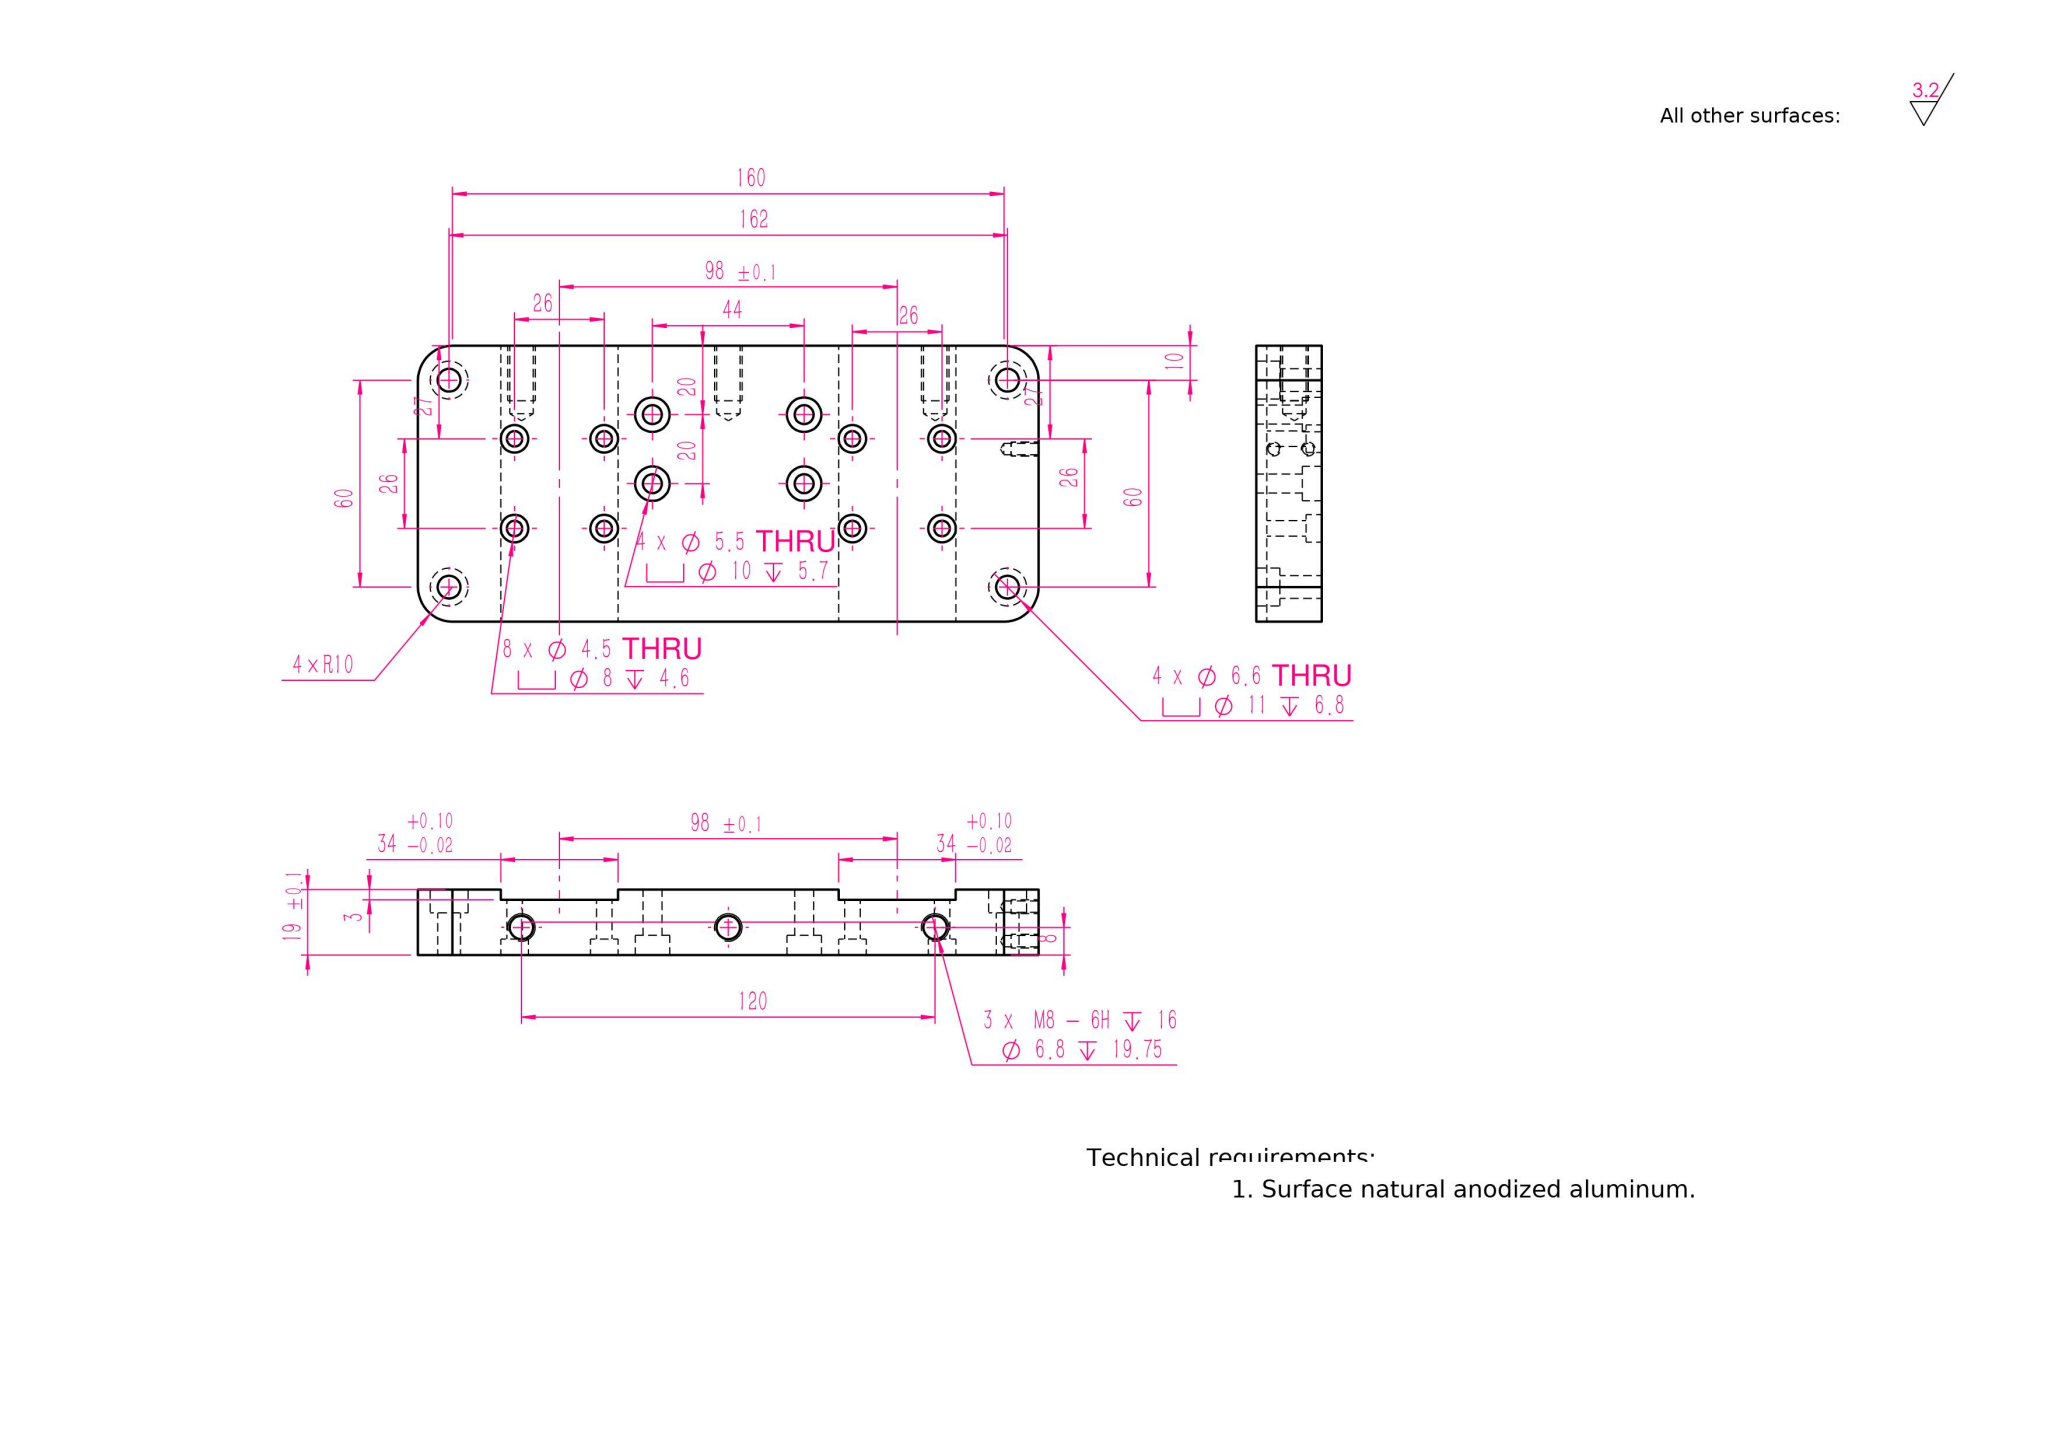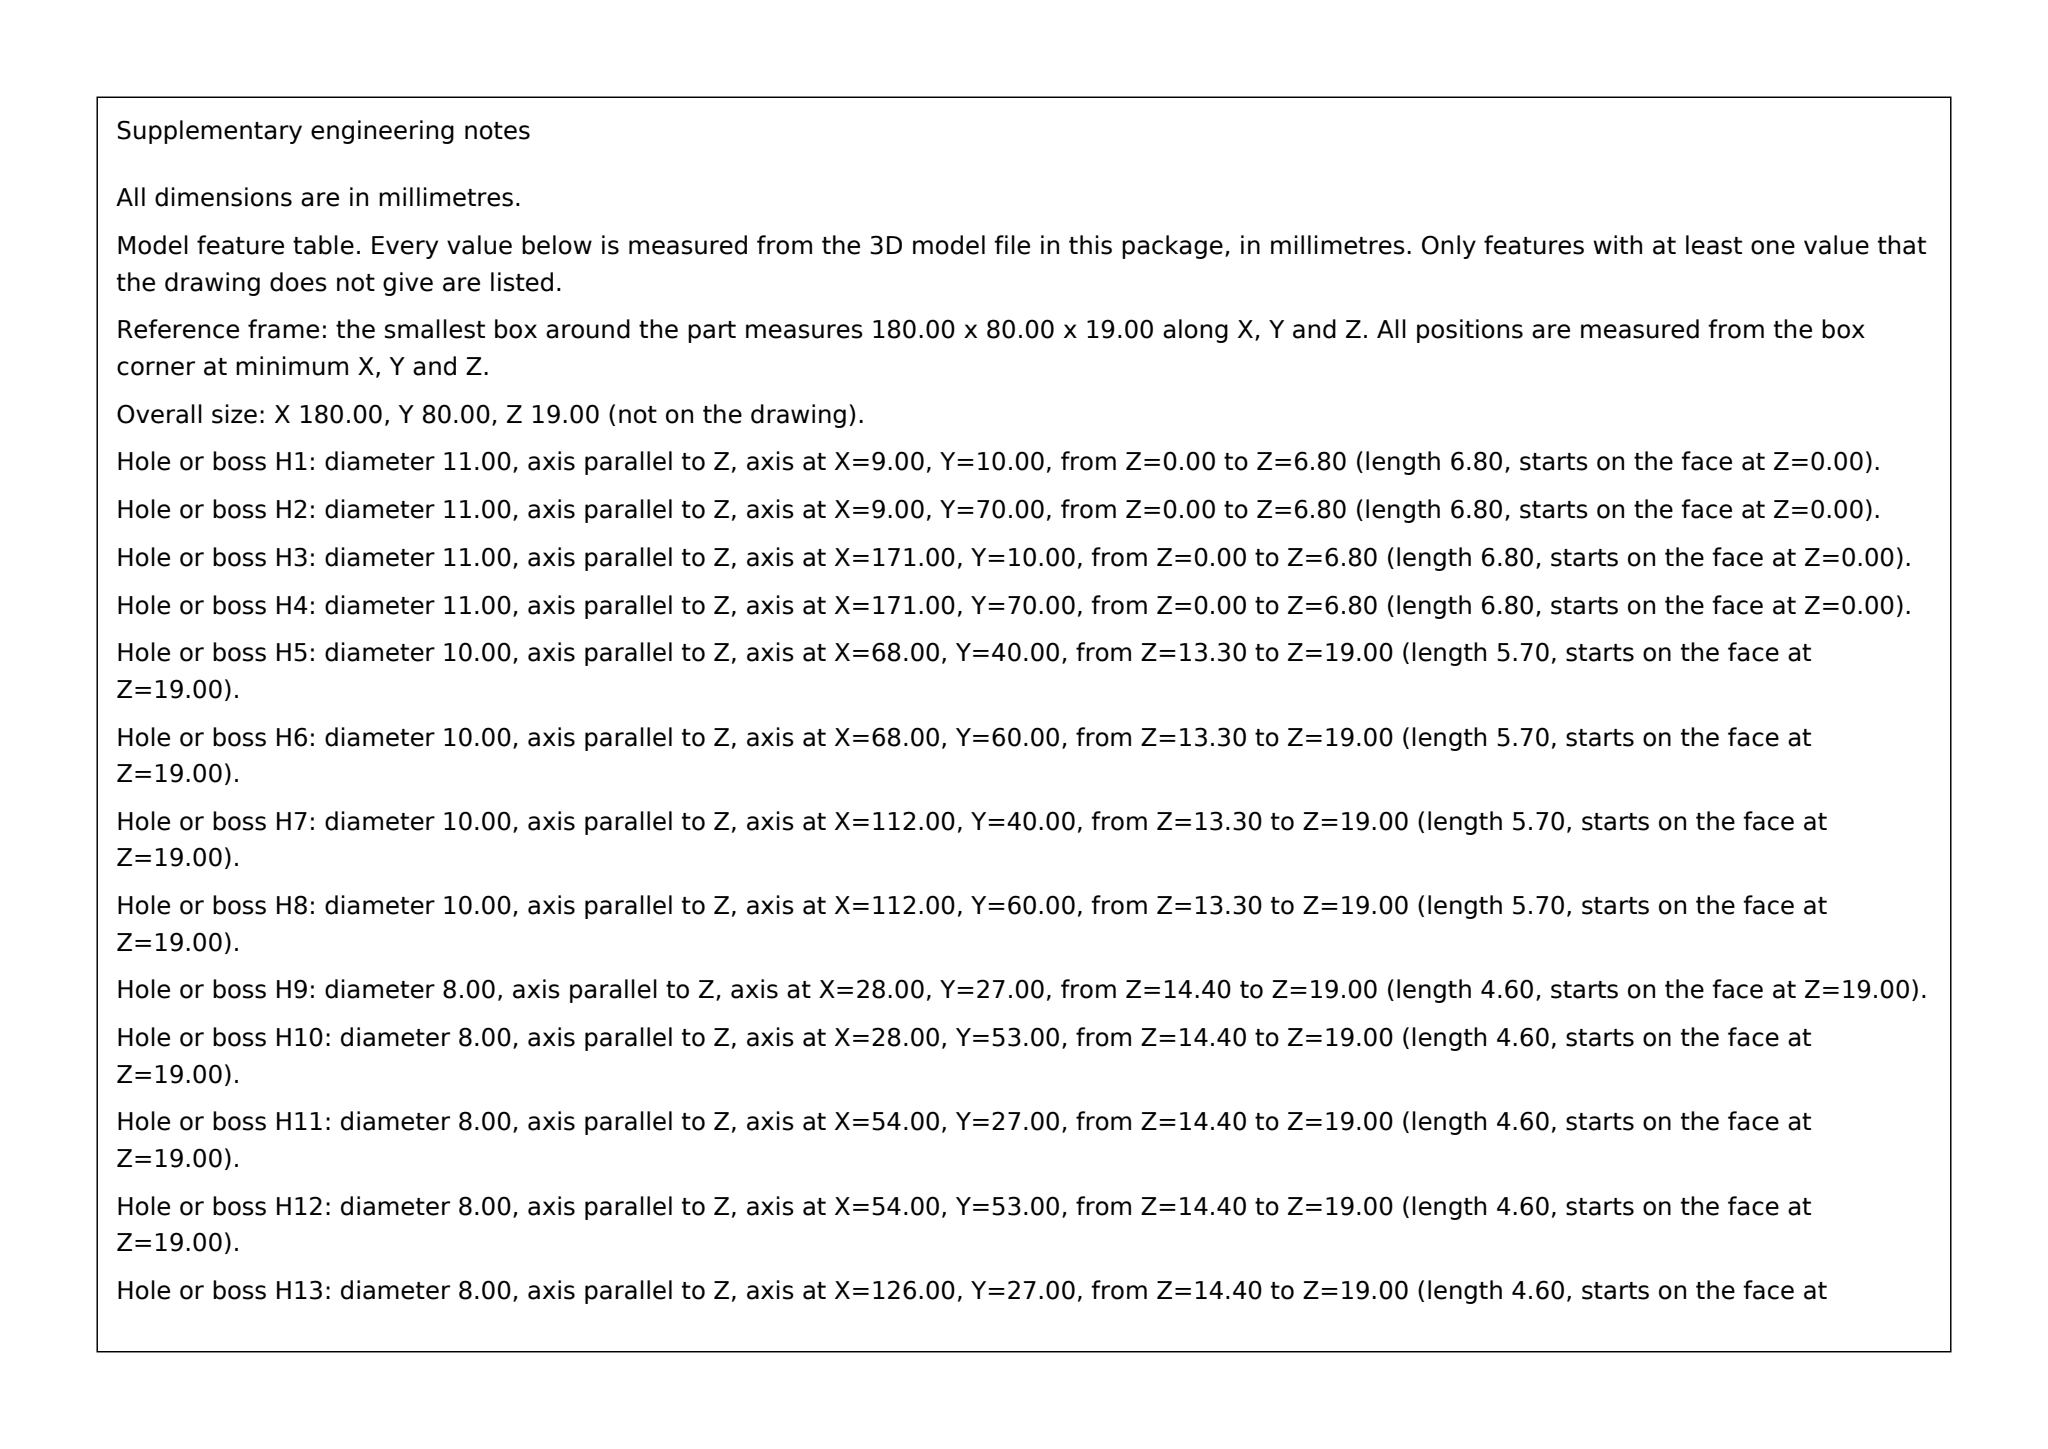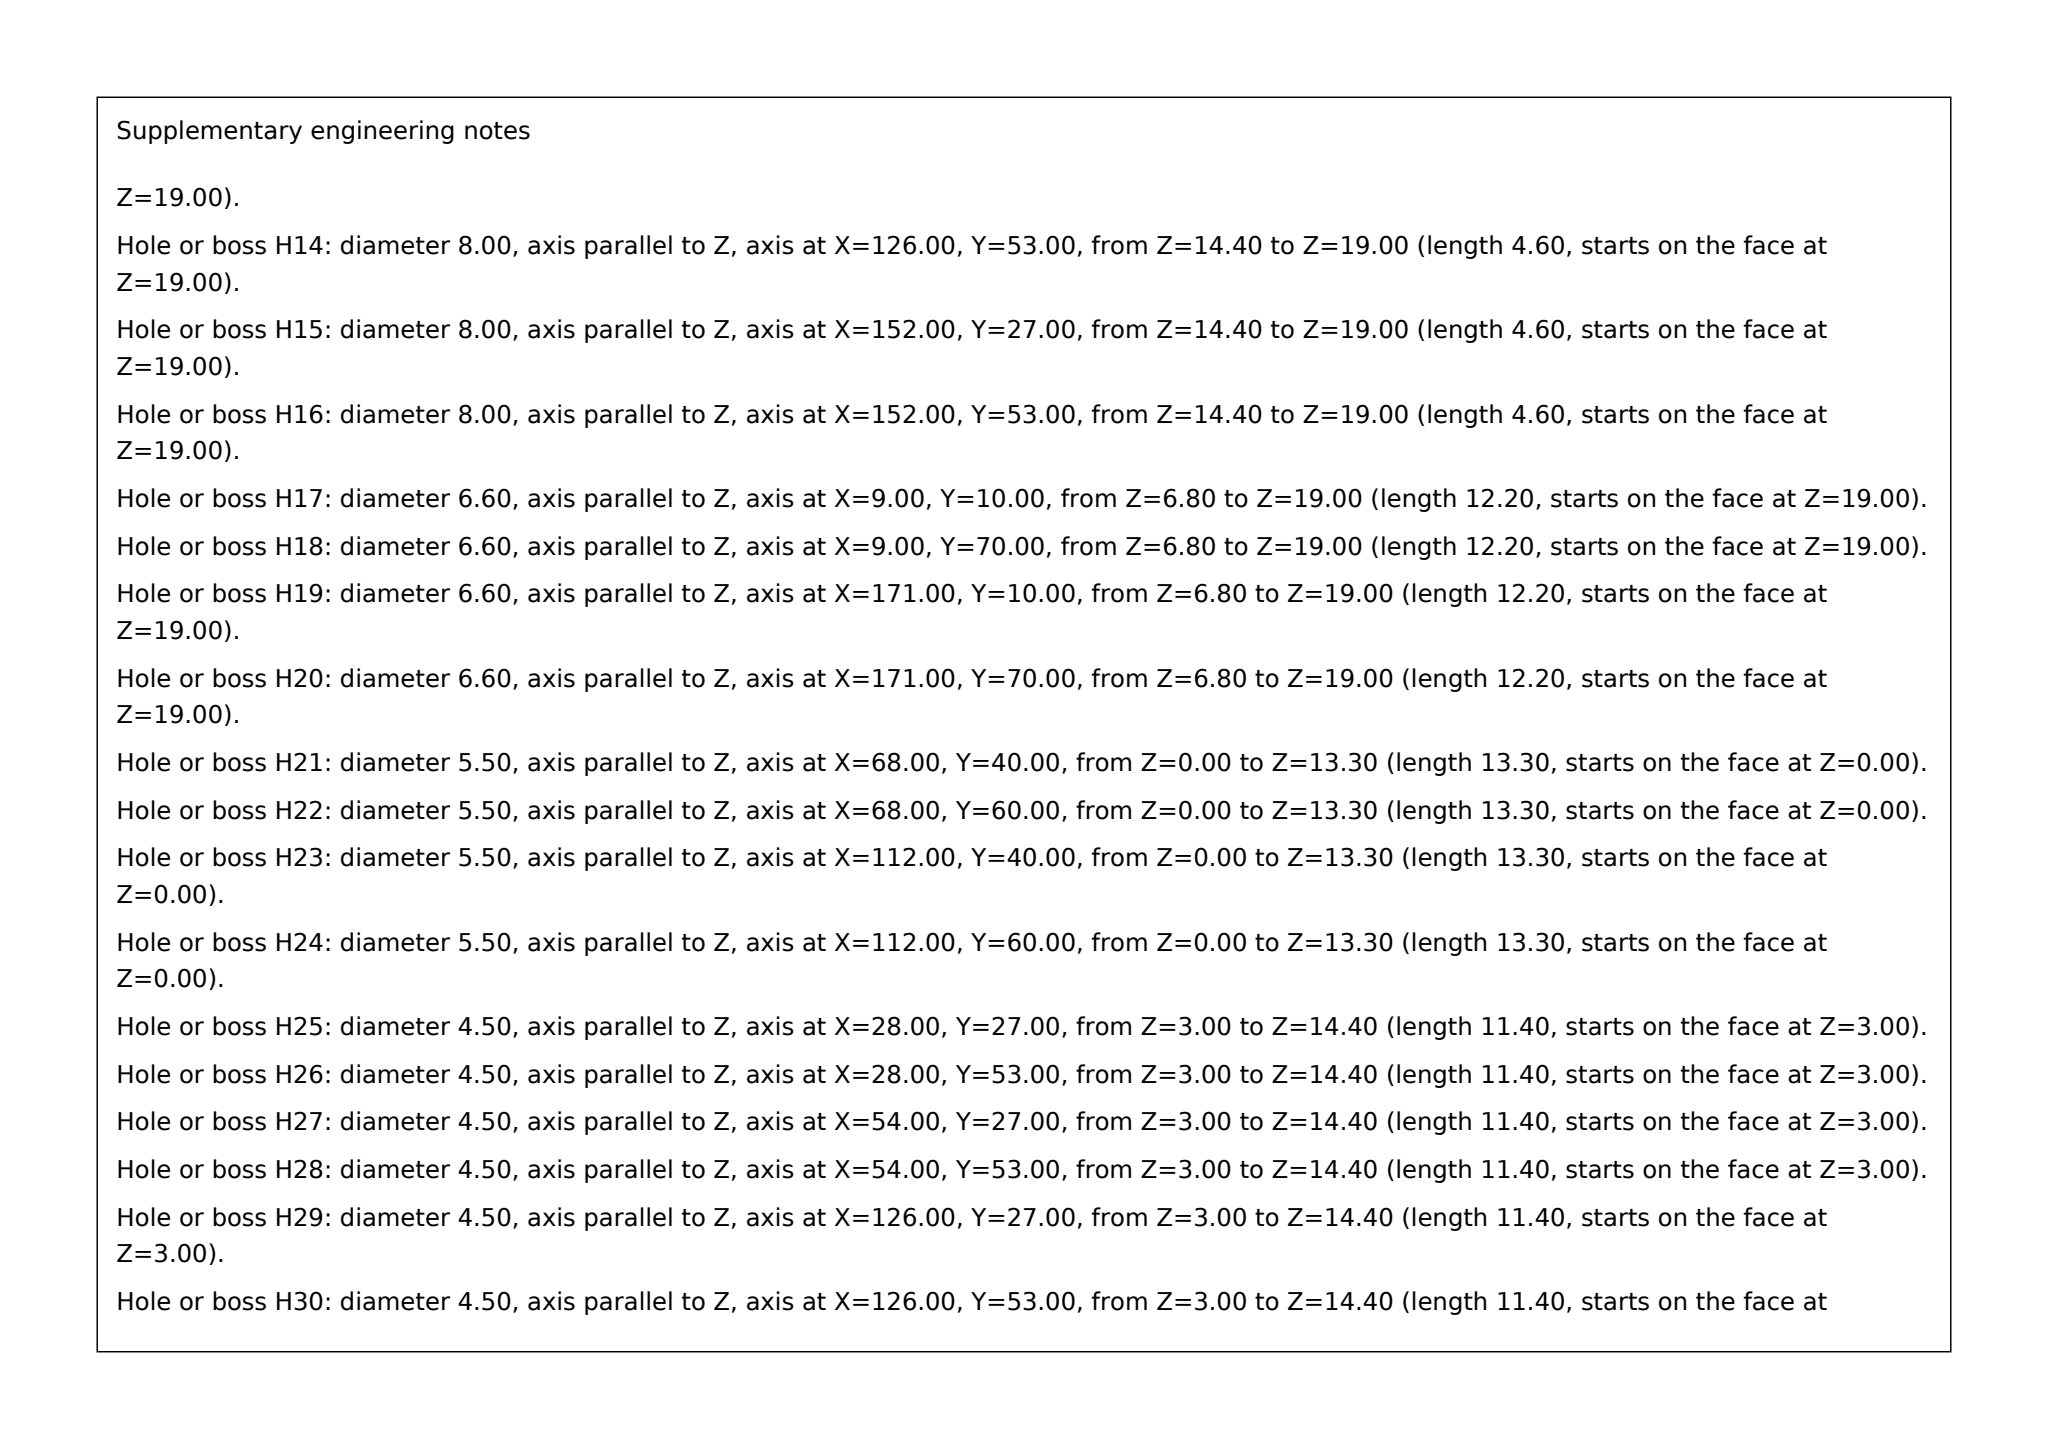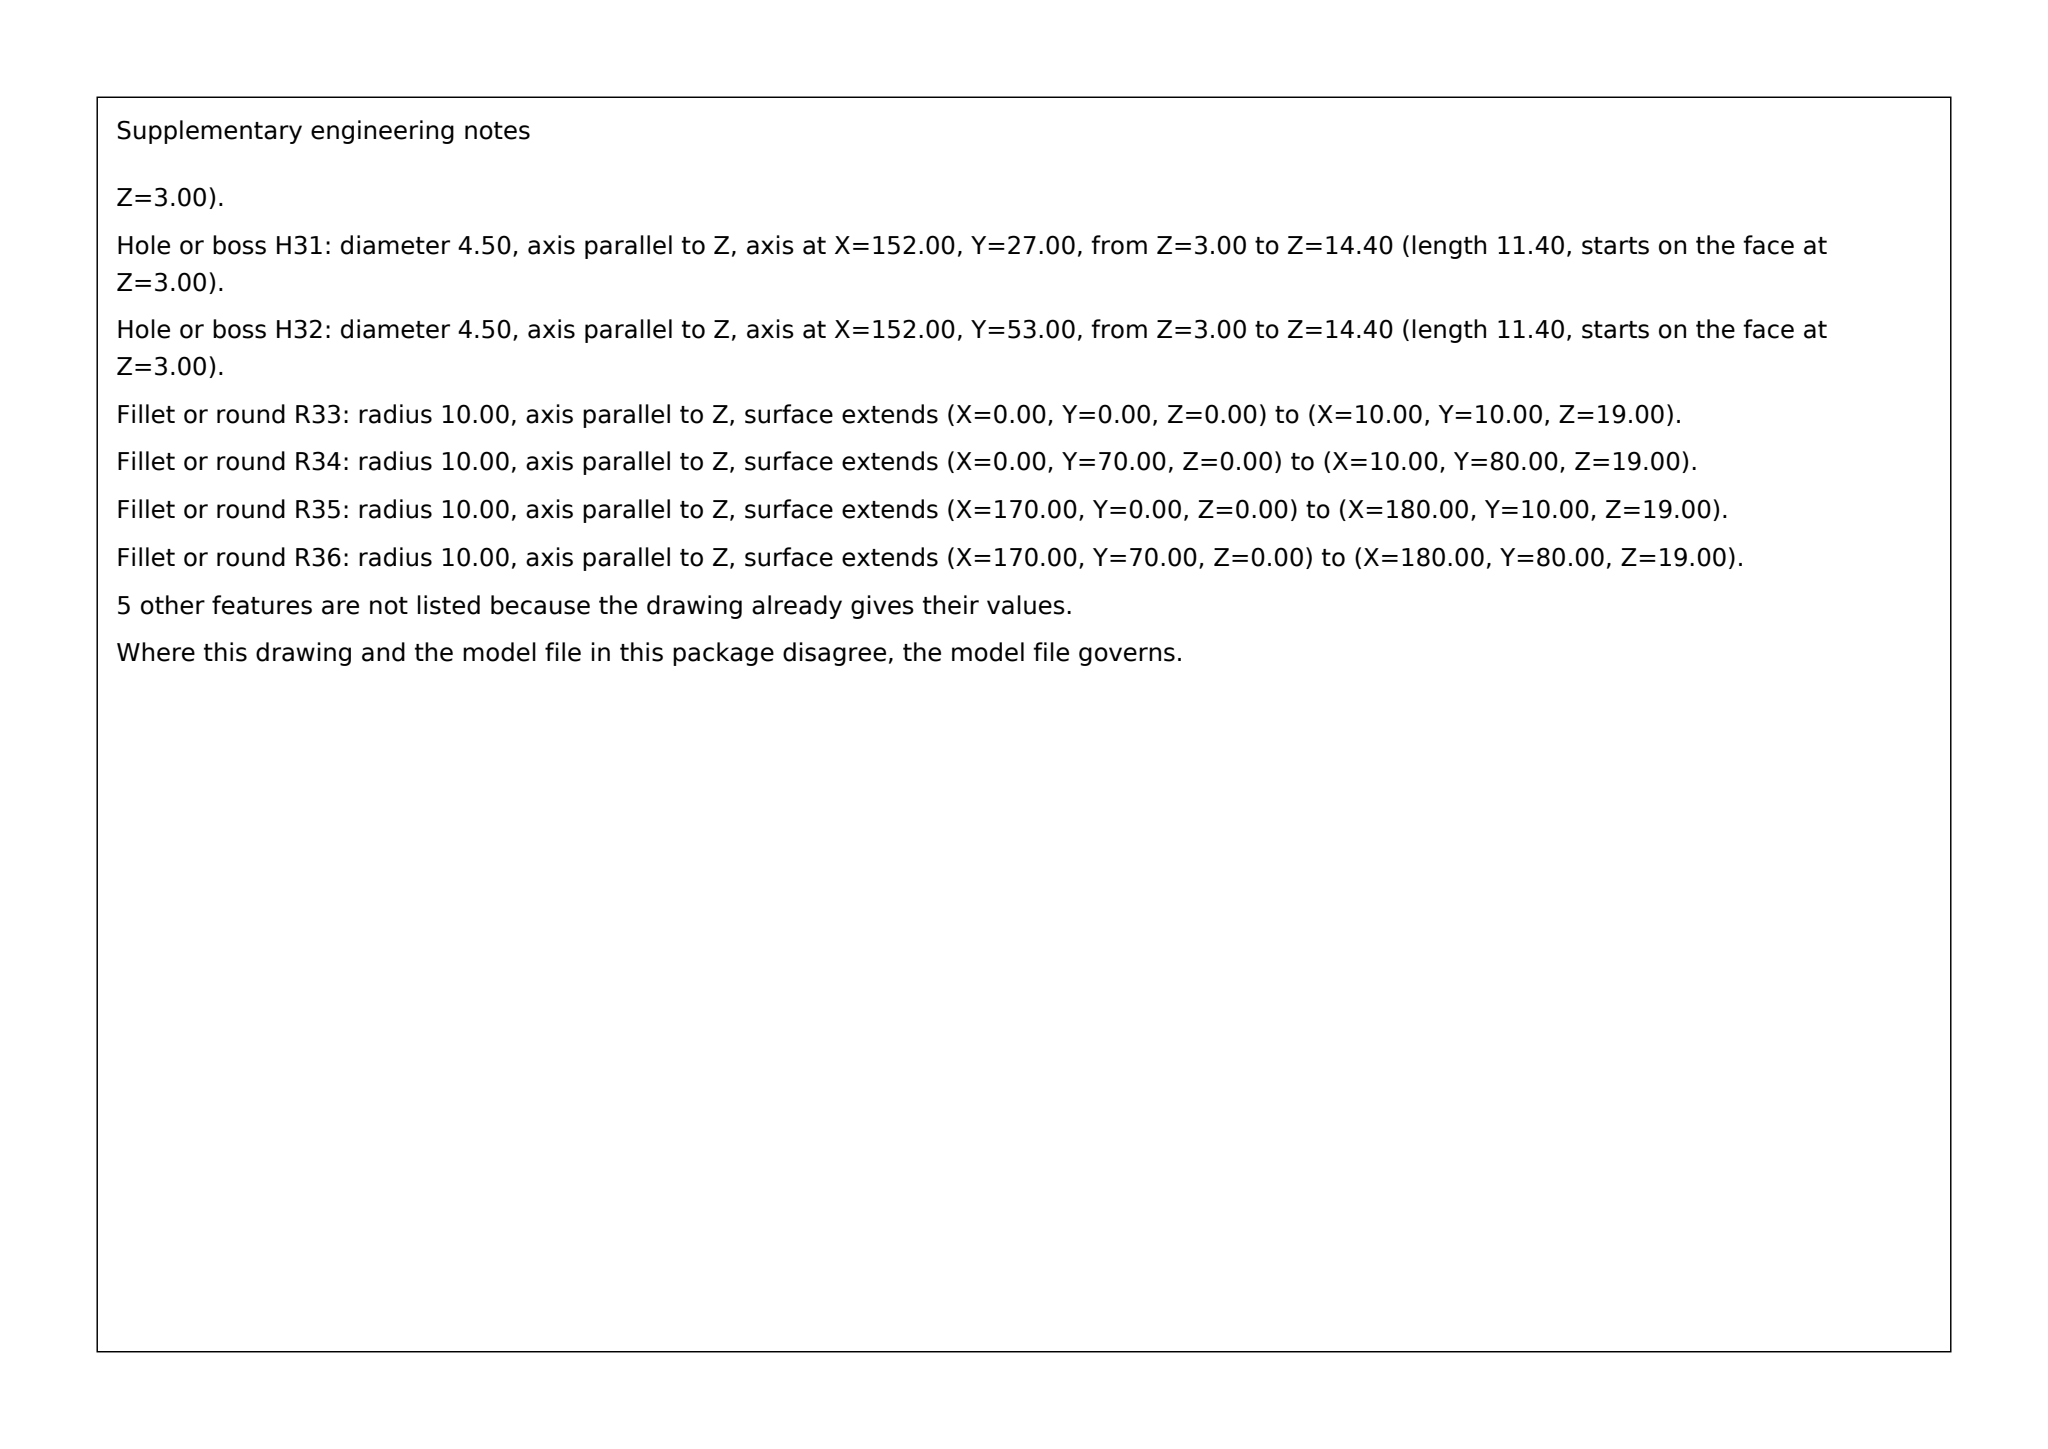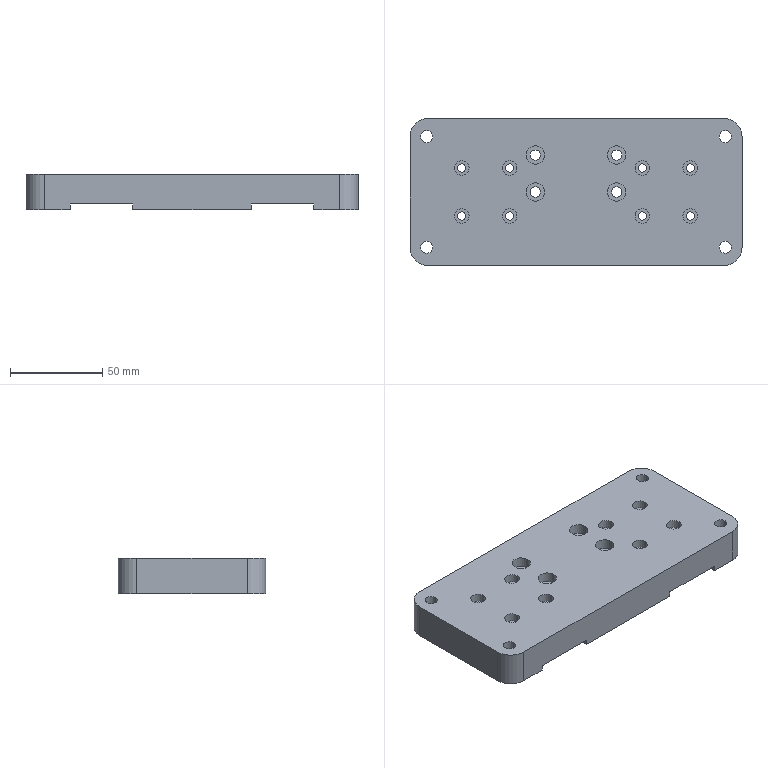Part | SolidWorks | mm | 1 solid | 118 faces | box 180 x 80 x 19 mm | volume 242635 mm3 | cylinder 78 | plane 30 | cone 10 | commonest cylinder face diameters 8 x16 4.5 x16 11 x8 6.6 x8 10 x8 5.5 x8 6.8 x6 3.3 x4
build123d program:
from build123d import *

# Parameters (mm, degrees)
SKETCH1_W                                            = 180
SKETCH1_H                                            = 80
BOSS_EXTRUDE1_DEPTH                                  = 9.5
SKETCH2_W                                            = 34
SKETCH2_H                                            = 3
CUT_EXTRUDE1_DEPTH                                   = 121.79
HOLE_SIZE_ACCORDING_TO_HEXAGON_SOCKET_HE_D           = 4.5
HOLE_SIZE_ACCORDING_TO_HEXAGON_SOCKET_HE_CBORE_D     = 8
HOLE_SIZE_ACCORDING_TO_HEXAGON_SOCKET_HE_CBORE_DEPTH = 4.6
HOLE_SIZE_ACCORDING_TO_HEXAGON_SOCKE_2_D             = 5.5
HOLE_SIZE_ACCORDING_TO_HEXAGON_SOCKE_2_CBORE_D       = 10
HOLE_SIZE_ACCORDING_TO_HEXAGON_SOCKE_2_CBORE_DEPTH   = 5.7
M8_TAPPED_HOLE1_D                                    = 6.8
M8_TAPPED_HOLE1_DEPTH                                = 19.75
M8_TAPPED_HOLE1_TIP                                  = 2.043
HOLE_SIZE_ACCORDING_TO_HEXAGON_SOCKE_3_D             = 6.6
HOLE_SIZE_ACCORDING_TO_HEXAGON_SOCKE_3_CBORE_D       = 11
HOLE_SIZE_ACCORDING_TO_HEXAGON_SOCKE_3_CBORE_DEPTH   = 6.8
M4_TAPPED_HOLE1_D                                    = 3.3
M4_TAPPED_HOLE1_DEPTH                                = 10.1
M4_TAPPED_HOLE1_TIP                                  = 0.9914
FILLET1_R                                            = 10


with BuildPart() as part:
    # Sketch1 → Boss-Extrude1 (new, symmetric)
    with BuildSketch(Plane.XY):
        with Locations((0, 40)):
            Rectangle(SKETCH1_W, SKETCH1_H)
    extrude(amount=BOSS_EXTRUDE1_DEPTH, both=True)

    # Sketch2 → Cut-Extrude1 (cut, through all)
    with BuildSketch(Plane(origin=(0, 80, 0), x_dir=(1, 0, 0), z_dir=(0, 1, 0))):
        with Locations((-49, 8)):
            Rectangle(SKETCH2_W, SKETCH2_H)
        with Locations((49, 8)):
            Rectangle(SKETCH2_W, SKETCH2_H)
    extrude(amount=-CUT_EXTRUDE1_DEPTH, mode=Mode.SUBTRACT)

    # Hole Size according to Hexagon Socket He (through all)
    with Locations(Plane.XY.offset(9.5)):
        with Locations((-62, 53), (-36, 53), (-62, 27), (-36, 27), (36, 27), (62, 27), (36, 53), (62, 53)):
            CounterBoreHole(HOLE_SIZE_ACCORDING_TO_HEXAGON_SOCKET_HE_D / 2, HOLE_SIZE_ACCORDING_TO_HEXAGON_SOCKET_HE_CBORE_D / 2, HOLE_SIZE_ACCORDING_TO_HEXAGON_SOCKET_HE_CBORE_DEPTH)

    # Hole Size according to Hexagon Socke 2 (through all)
    with Locations(Plane.XY.offset(9.5)):
        with Locations((-22, 60), (-22, 40), (22, 40), (22, 60)):
            CounterBoreHole(HOLE_SIZE_ACCORDING_TO_HEXAGON_SOCKE_2_D / 2, HOLE_SIZE_ACCORDING_TO_HEXAGON_SOCKE_2_CBORE_D / 2, HOLE_SIZE_ACCORDING_TO_HEXAGON_SOCKE_2_CBORE_DEPTH)

    # M8 Tapped Hole1
    with Locations(Plane(origin=(0, 80, 0), x_dir=(1, 0, 0), z_dir=(0, 1, 0))):
        with Locations((-60, -1.5), (0, -1.5), (60, -1.5)):
            Hole(M8_TAPPED_HOLE1_D / 2, depth=M8_TAPPED_HOLE1_DEPTH)
            with Locations((0, 0, -(M8_TAPPED_HOLE1_DEPTH + M8_TAPPED_HOLE1_TIP / 2))):  # 118° drill point
                Cone(0, M8_TAPPED_HOLE1_D / 2, M8_TAPPED_HOLE1_TIP, mode=Mode.SUBTRACT)

    # Hole Size according to Hexagon Socke 3 (through all)
    with Locations(Plane(origin=(0, 0, -9.5), x_dir=(-1, 0, 0), z_dir=(0, 0, -1))):
        with Locations((-81, 70), (-81, 10), (81, 10), (81, 70)):
            CounterBoreHole(HOLE_SIZE_ACCORDING_TO_HEXAGON_SOCKE_3_D / 2, HOLE_SIZE_ACCORDING_TO_HEXAGON_SOCKE_3_CBORE_D / 2, HOLE_SIZE_ACCORDING_TO_HEXAGON_SOCKE_3_CBORE_DEPTH)

    # M4 Tapped Hole1
    with Locations(Plane(origin=(90, 0, 0), x_dir=(0, 0, -1), z_dir=(1, 0, 0))):
        with Locations((4.5, 50), (-5.5, 50)):
            Hole(M4_TAPPED_HOLE1_D / 2, depth=M4_TAPPED_HOLE1_DEPTH)
            with Locations((0, 0, -(M4_TAPPED_HOLE1_DEPTH + M4_TAPPED_HOLE1_TIP / 2))):  # 118° drill point
                Cone(0, M4_TAPPED_HOLE1_D / 2, M4_TAPPED_HOLE1_TIP, mode=Mode.SUBTRACT)

    # Fillet1
    fillet1_edges = [part.edges().sort_by_distance(p)[0] for p in [
        (-90, 80, 0),
        (90, 80, 0),
        (90, 0, 0),
        (-90, 0, 0),
    ]]
    fillet(fillet1_edges, radius=FILLET1_R)


solid = part.part